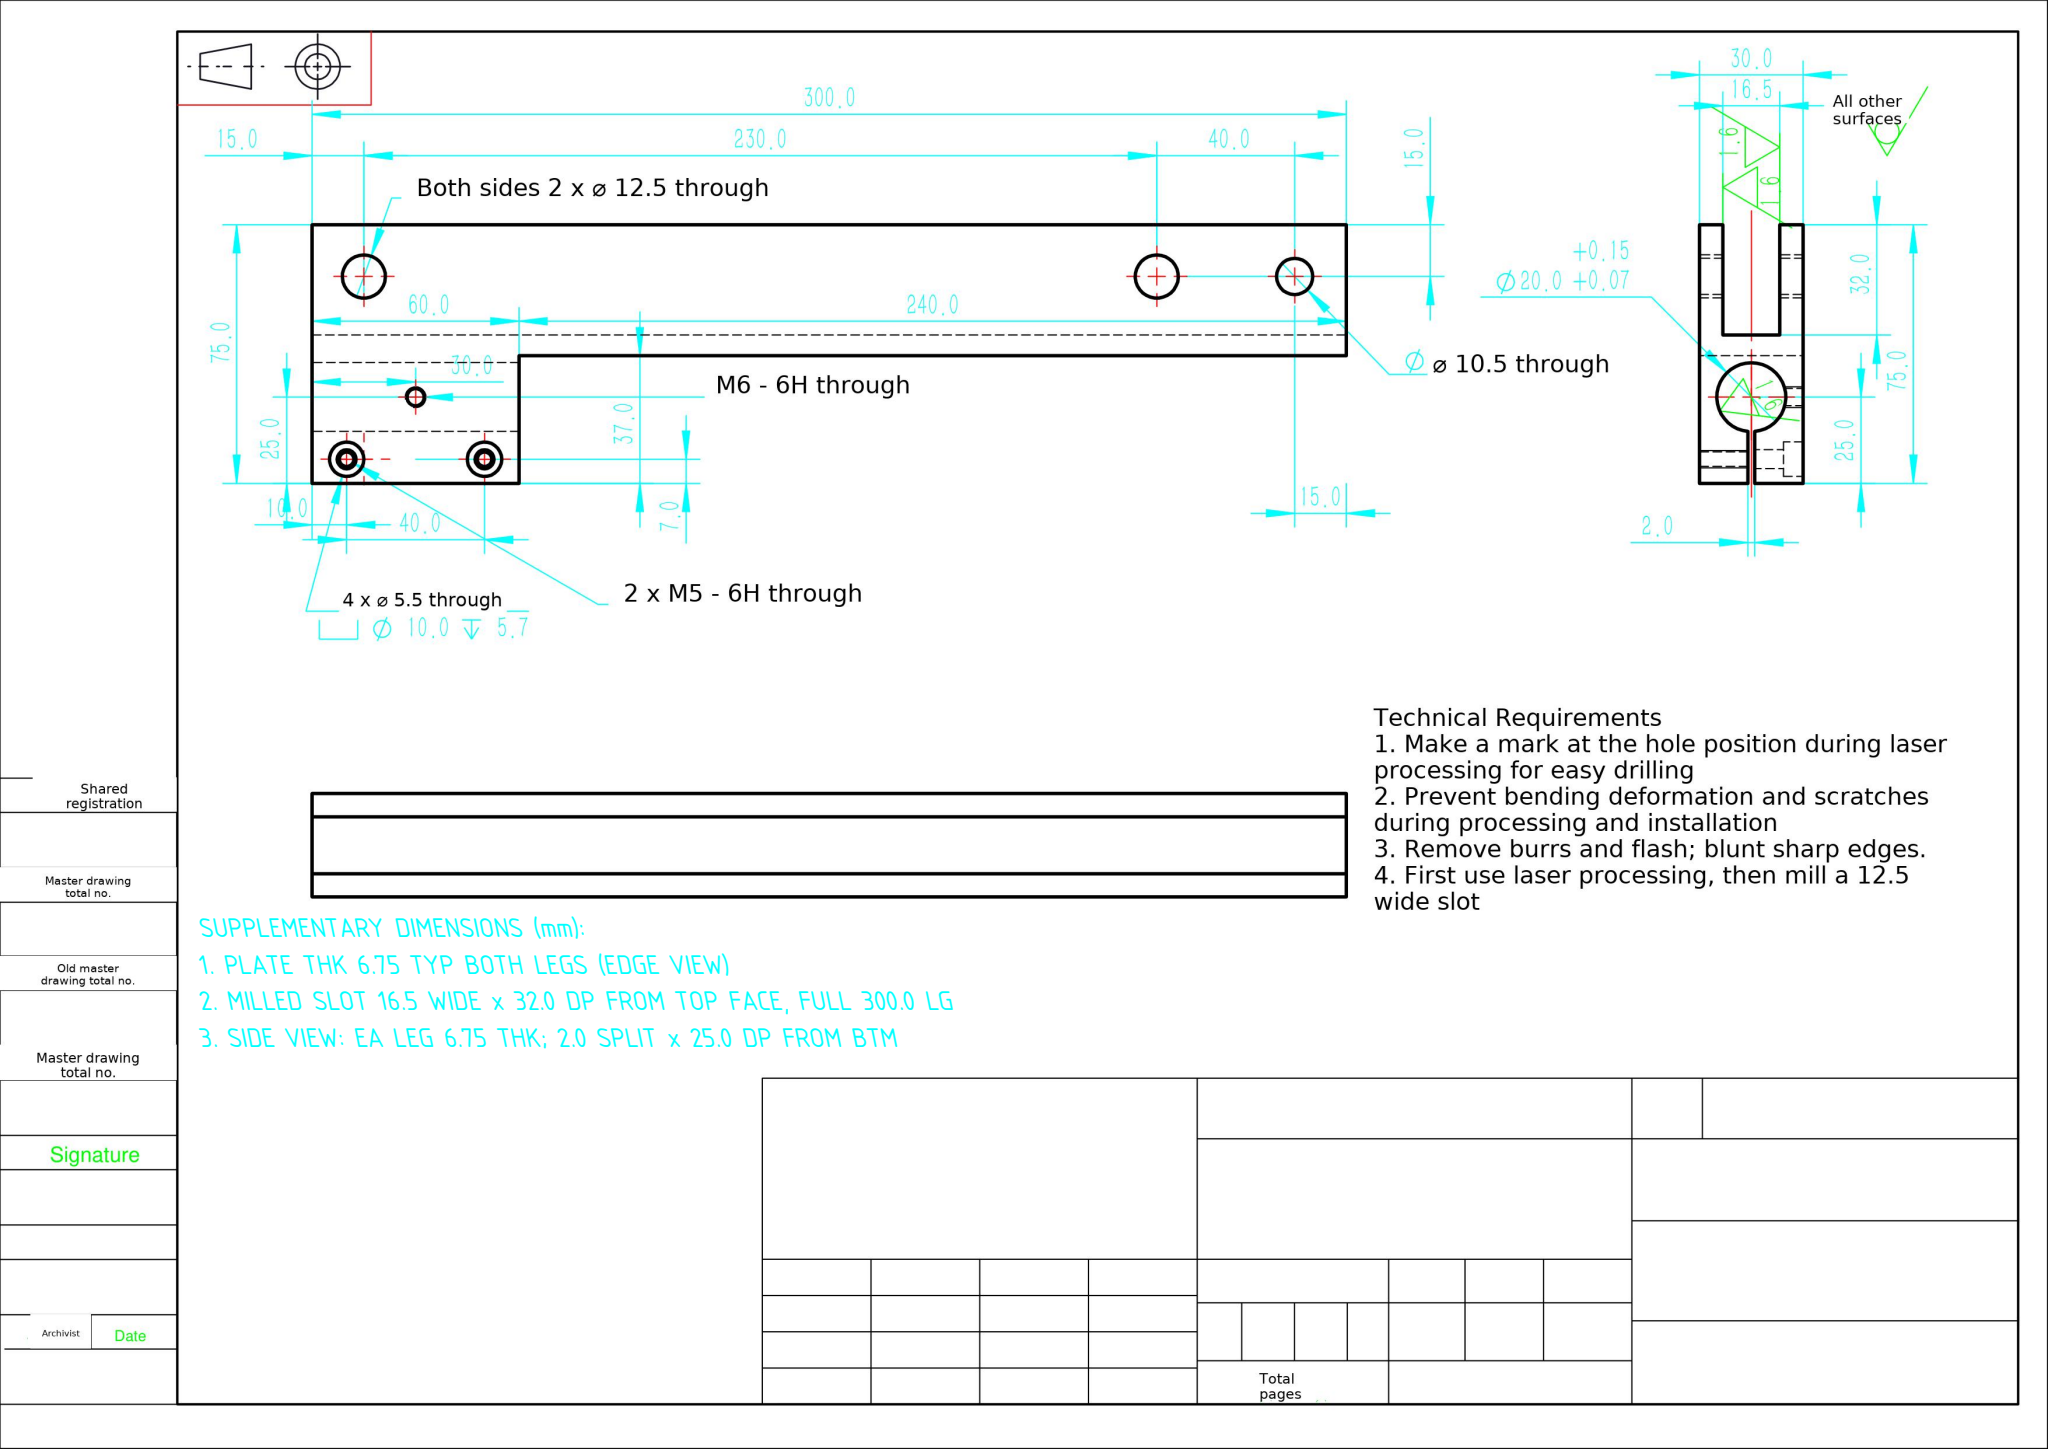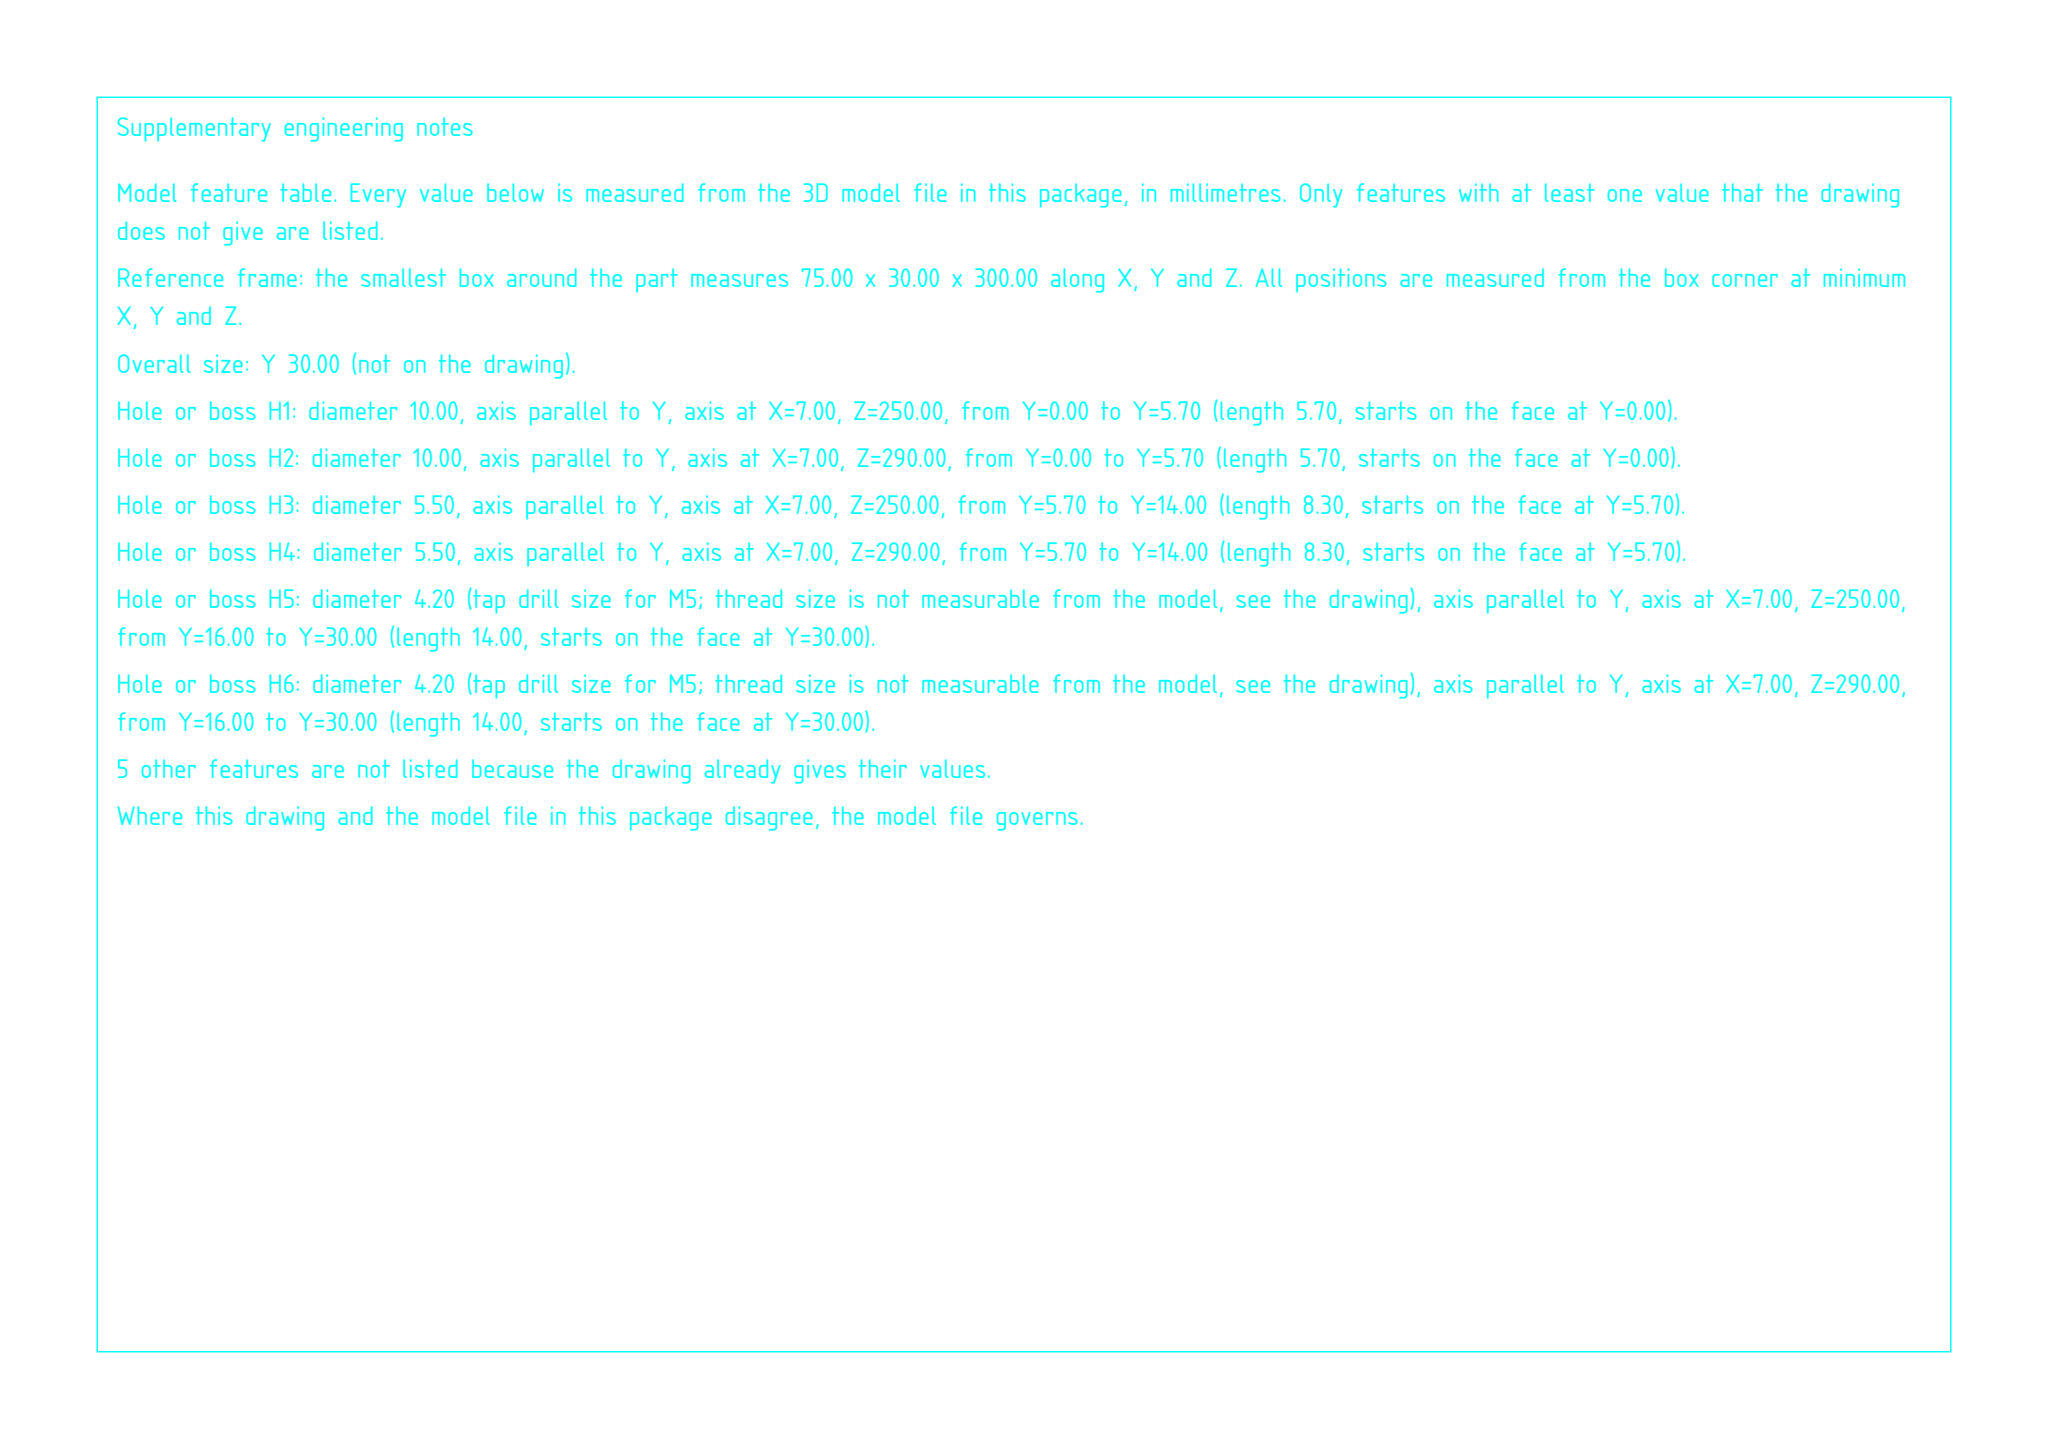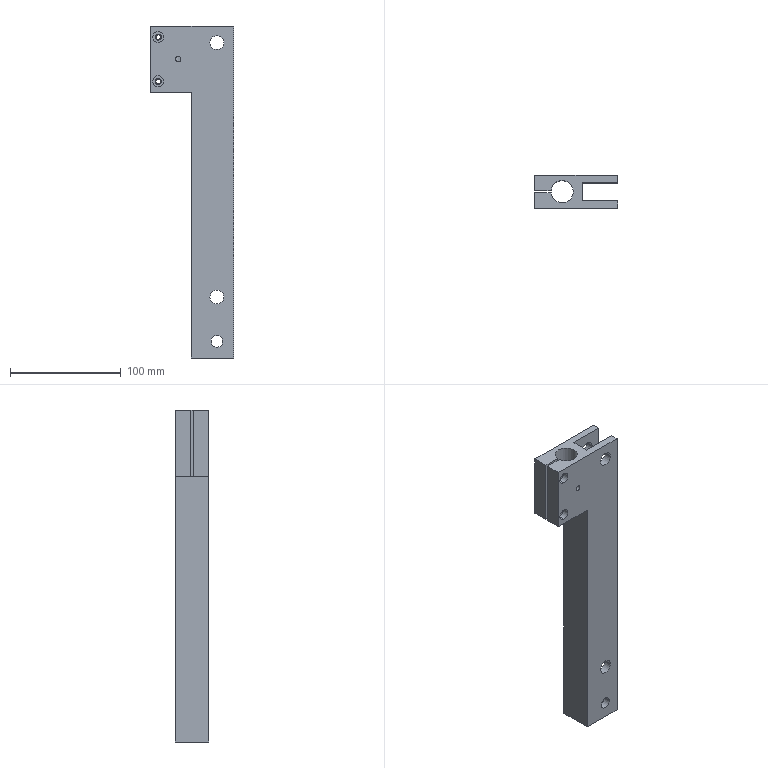Part | SolidWorks | mm | 1 solid | 44 faces | box 75 x 30 x 300 mm | volume 223289 mm3 | cylinder 27 | plane 17 | commonest cylinder face diameters 12.5 x8 4.2 x4 10 x4 5.5 x4 10.5 x4 5 x2 20 x1